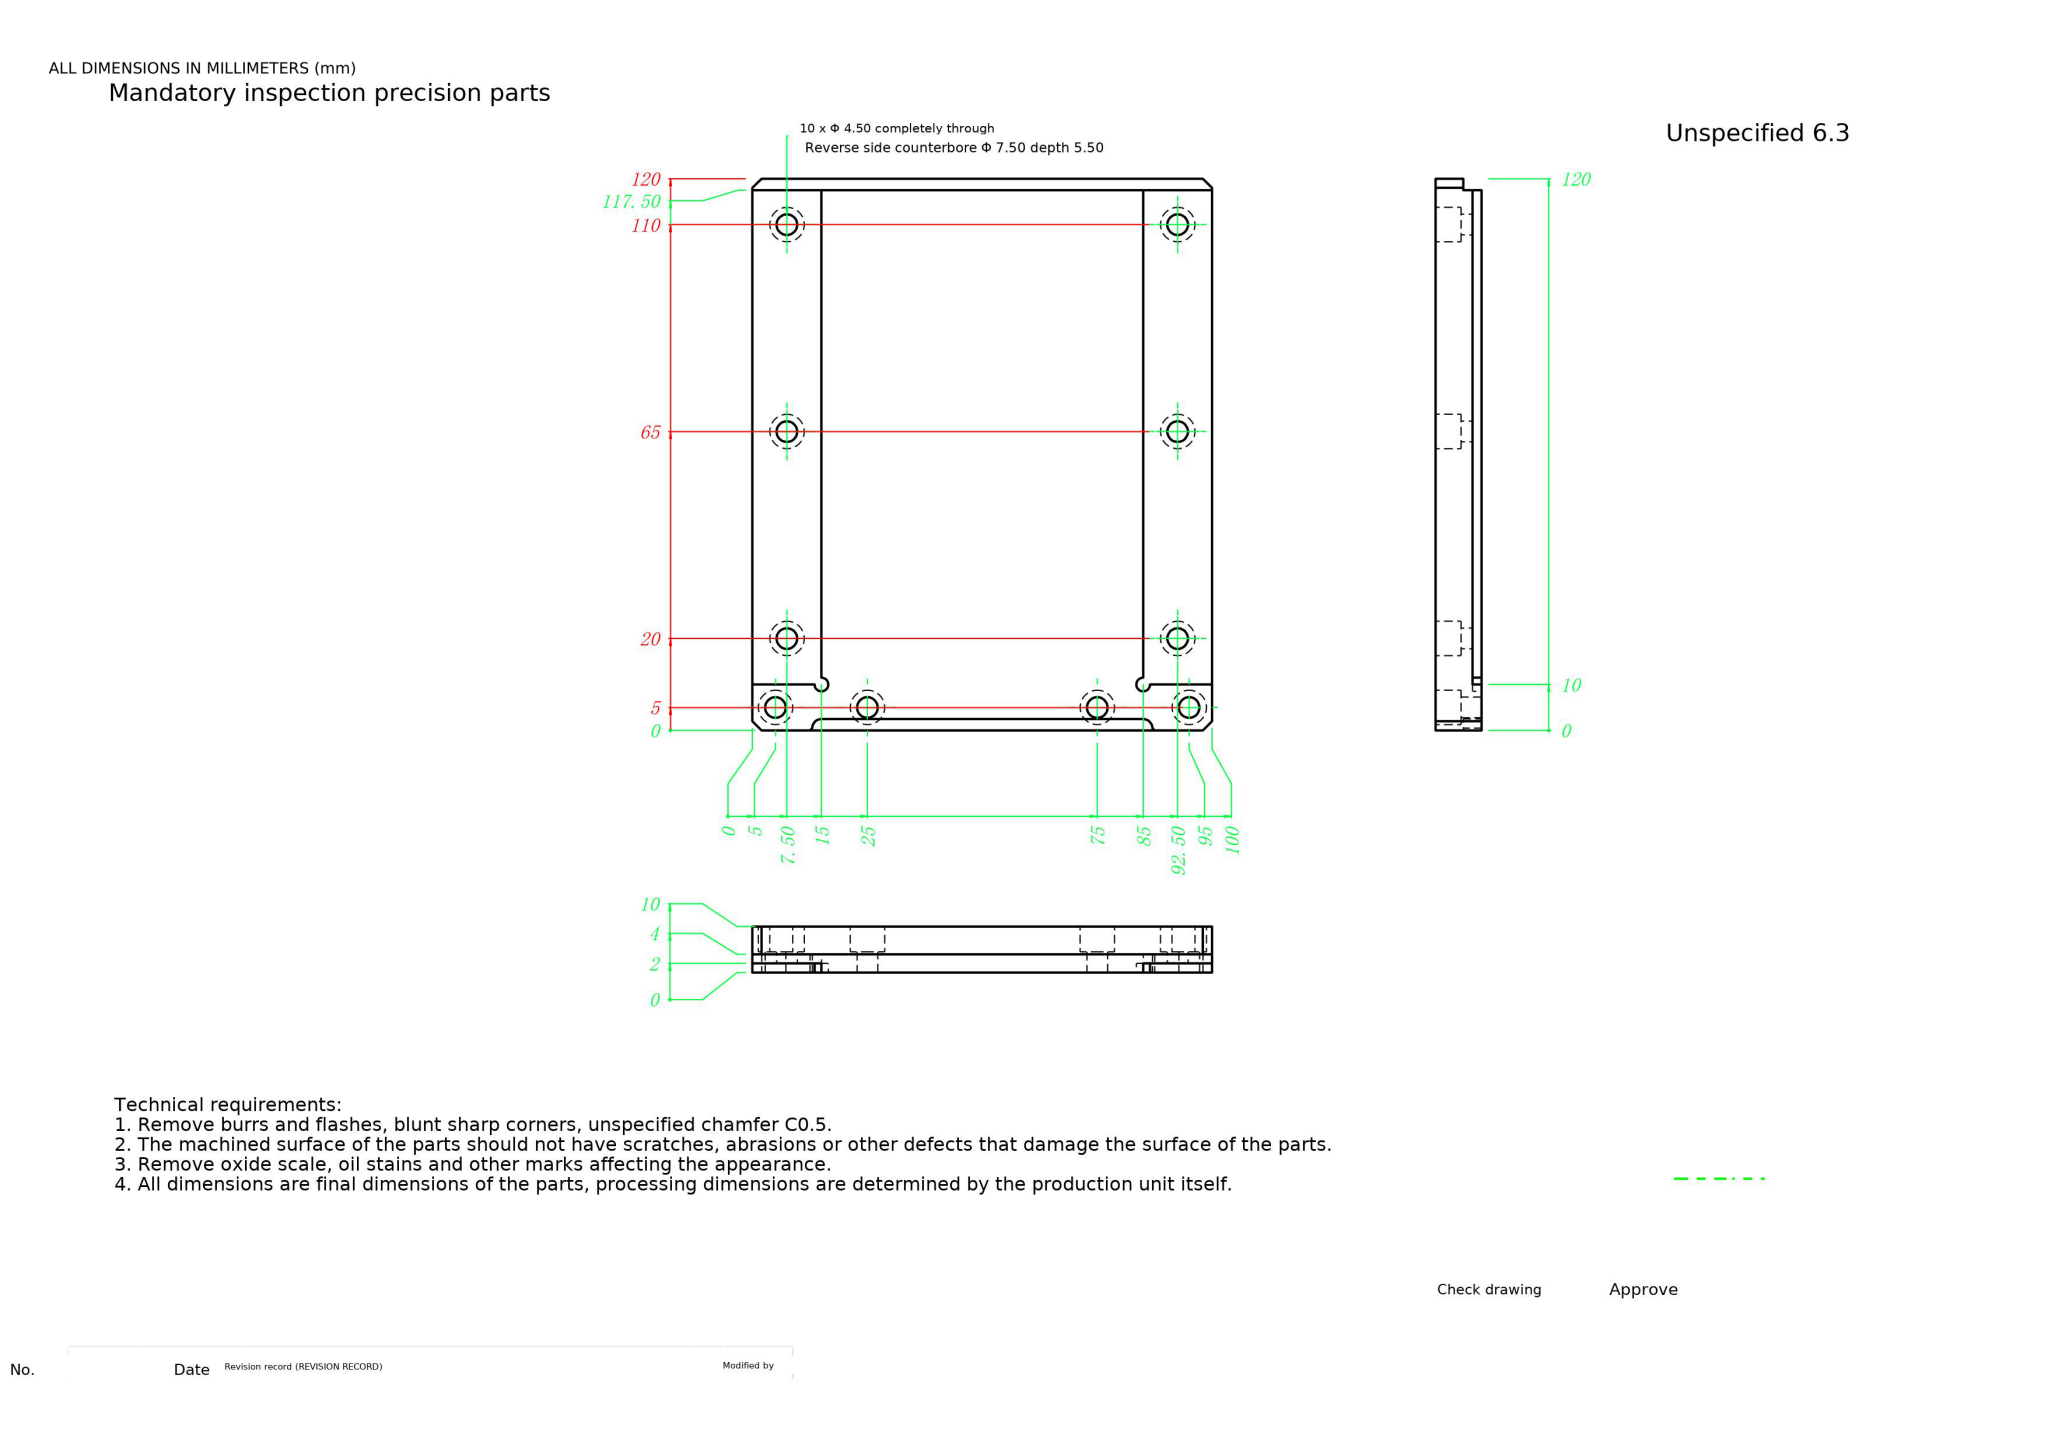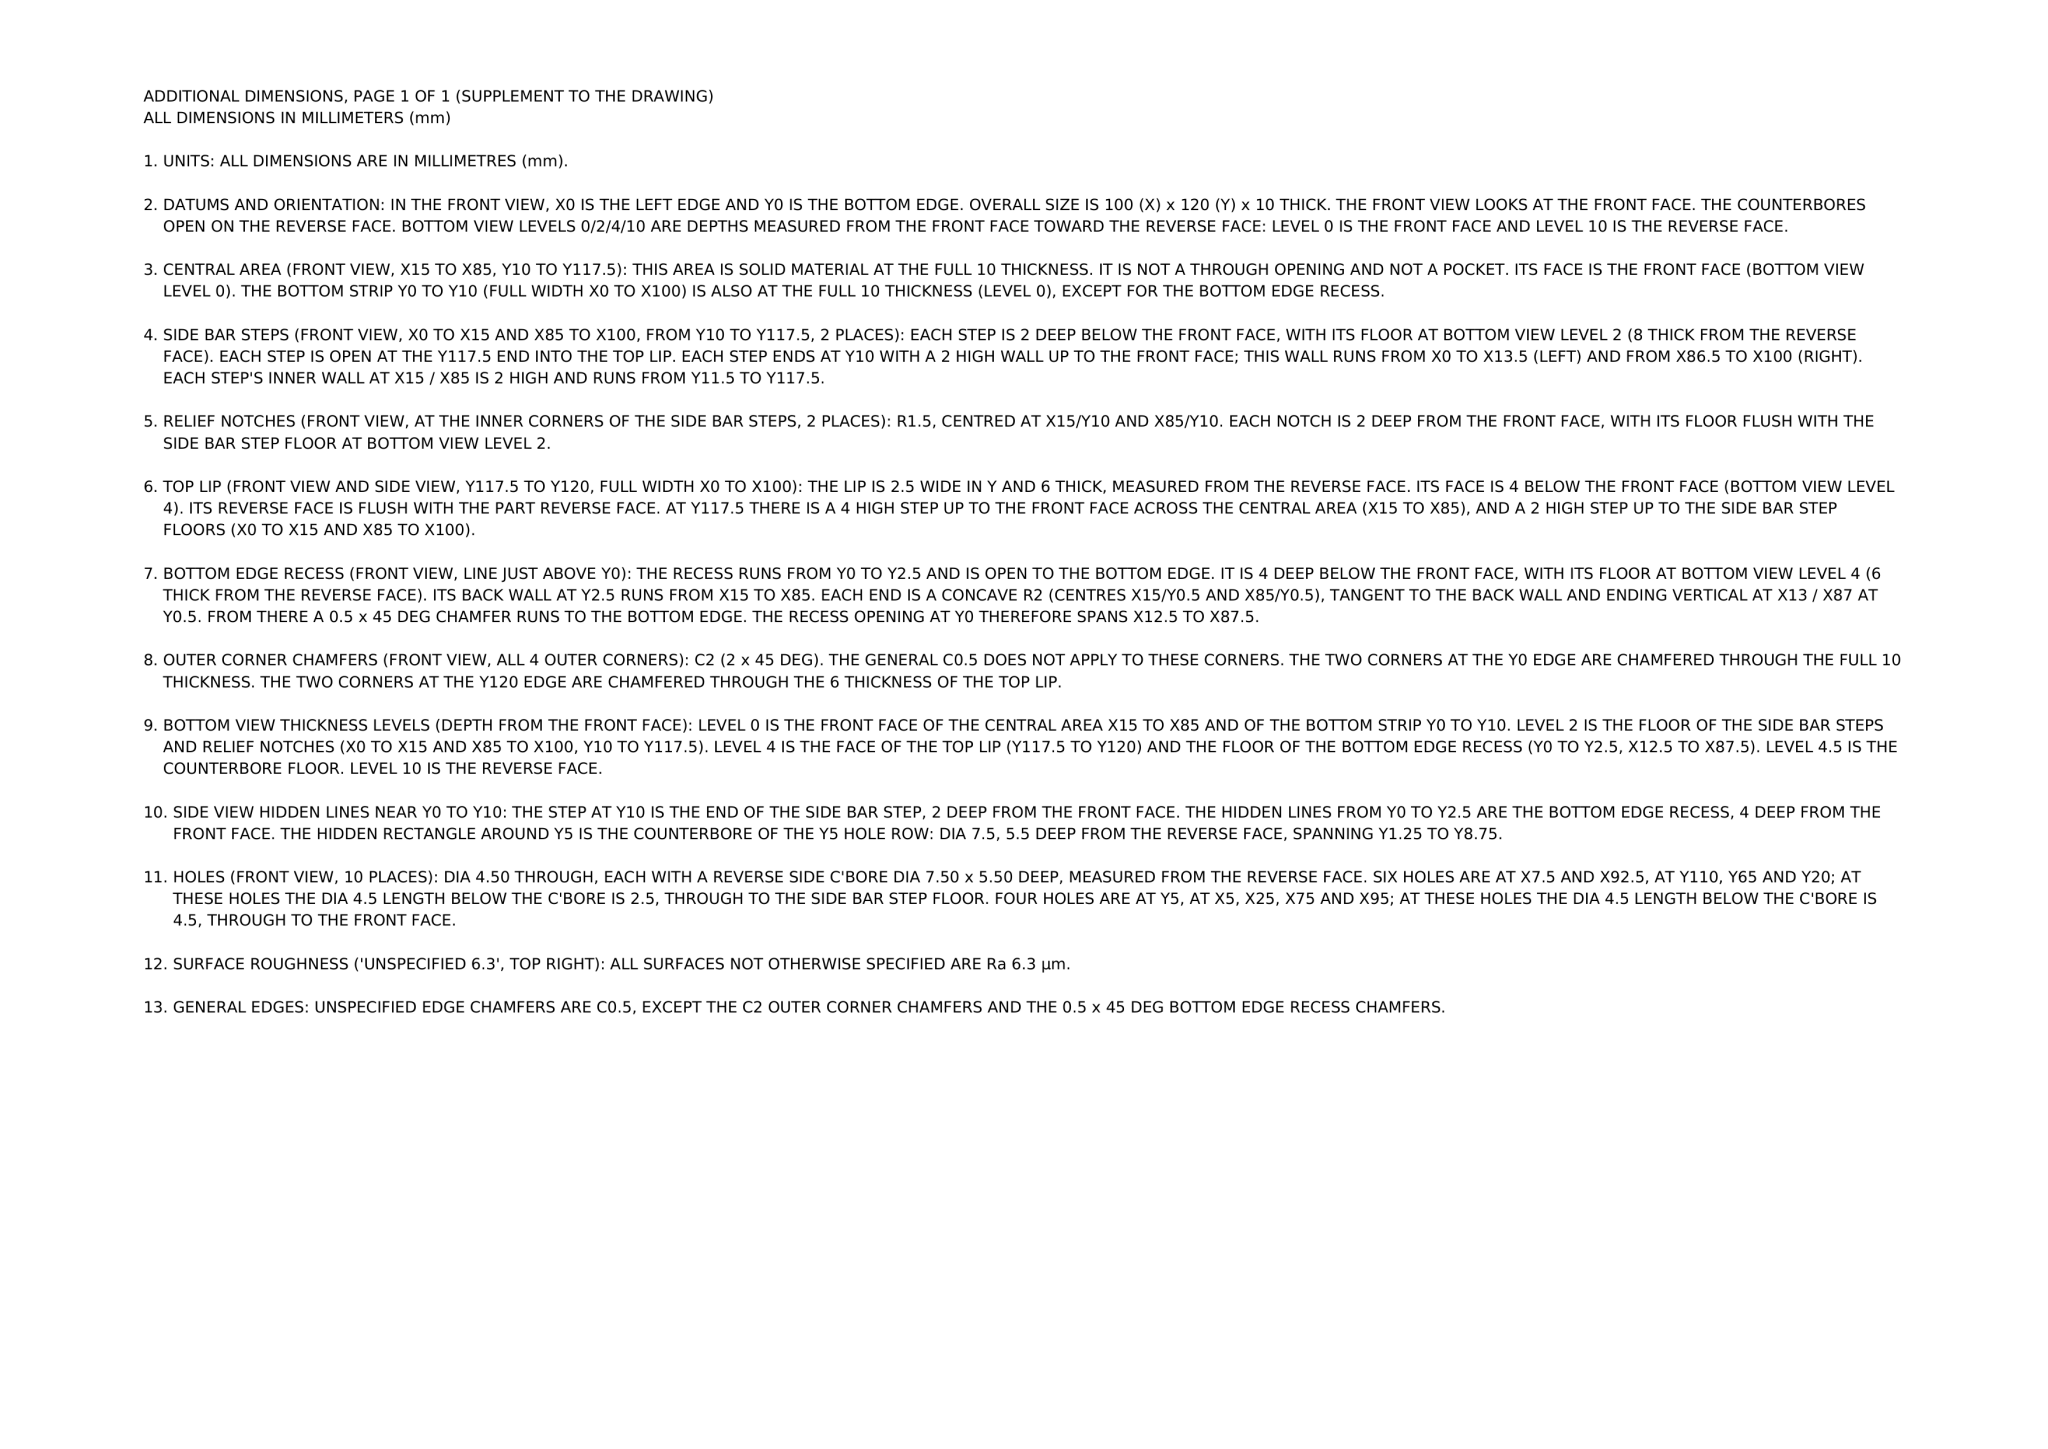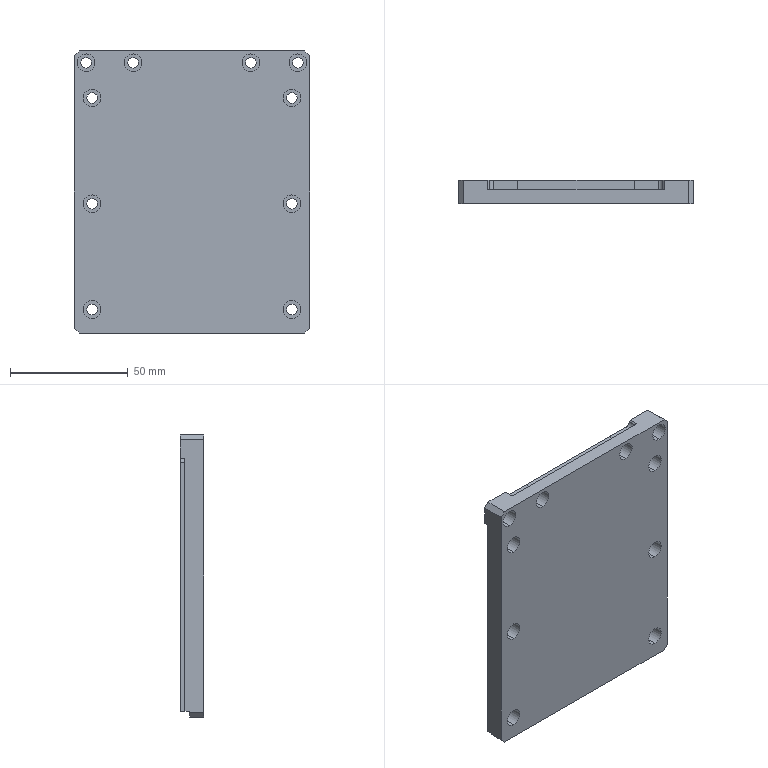Part | NX | mm | 1 solid | 78 faces | box 100 x 10 x 120 mm | volume 108776 mm3 | cylinder 46 | plane 32 | commonest cylinder face diameters 7.5 x20 4.5 x20 3 x4 4 x2